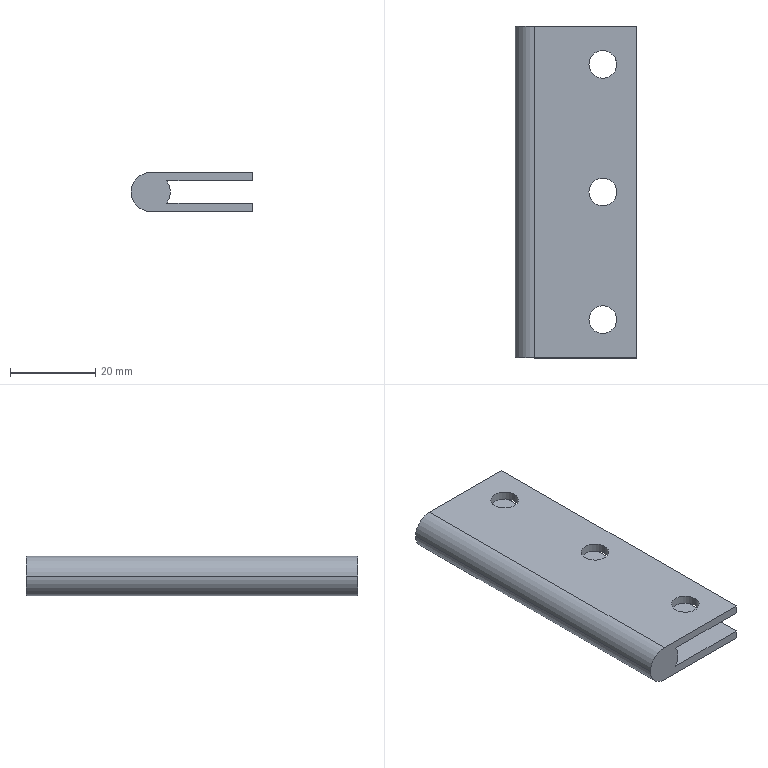Component | SolidWorks | SYM0671-81-200-1_SYMA1-51a_mis_shhpsk6-3-1 | 1 solid | 23 faces | box 28.6 x 78 x 9.2 mm | volume 11443 mm3 | cylinder 15 | plane 8 | commonest cylinder face diameters 6.5 x12 9.2 x3
build123d program:
from build123d import *

# Parameters (mm, degrees)
EXTRUDE1_DEPTH     = 39
SKETCH2_R          = 3.25
CUT_EXTRUDE1_DEPTH = 47.023
LPATTERN1_COUNT    = 3
LPATTERN1_PITCH    = 30


with BuildPart() as part:
    # Sketch1 → Extrude1 (new, symmetric)
    with BuildSketch(Plane(origin=(0, 0, 0), x_dir=(1, 0, 0), z_dir=(0, 1, 0))):
        with BuildLine():
            Line((-4.6, 0), (-4.6, -24))
            Line((-4.6, -24), (-2.6, -24))
            Line((-2.6, -24), (-2.6, -3.795))
            ThreePointArc((-2.6, -3.795), (0, -4.6), (2.6, -3.795))
            Line((2.6, -3.795), (2.6, -24))
            Line((2.6, -24), (4.6, -24))
            Line((4.6, -24), (4.6, 0))
            ThreePointArc((4.6, 0), (0, 4.6), (-4.6, 0))
        make_face()
    extrude(amount=EXTRUDE1_DEPTH, both=True)

    # Sketch2 → Cut-Extrude1 (cut, symmetric)
    with BuildSketch(Plane(origin=(0, 0, 0), x_dir=(0, 0, -1), z_dir=(1, 0, 0))):
        with Locations((-16, 30)):
            Circle(SKETCH2_R)
    cut_extrude1 = extrude(amount=CUT_EXTRUDE1_DEPTH, both=True, mode=Mode.SUBTRACT)

    # LPattern1: Cut-Extrude1 ×3
    with Locations(*[(0, -i * LPATTERN1_PITCH, 0) for i in range(1, LPATTERN1_COUNT)]):
        add(cut_extrude1, mode=Mode.SUBTRACT)


solid = part.part

# Placed as in the assembly
solid = solid.moved(Location((-402.749, 333.143, 1035.118), (0, 90, 0)))
STEP:
#1=COLOUR_RGB('',0.7922,0.8196,0.9333);
#2=FILL_AREA_STYLE_COLOUR('',#1);
#3=FILL_AREA_STYLE('',(#2));
#4=SURFACE_STYLE_FILL_AREA(#3);
#5=SURFACE_SIDE_STYLE('',(#4));
#6=SURFACE_STYLE_USAGE(.BOTH.,#5);
#7=PRESENTATION_STYLE_ASSIGNMENT((#6));
#8=CARTESIAN_POINT('',(-15.098,11.935,40.934));
#9=VERTEX_POINT('',#8);
#10=CARTESIAN_POINT('',(-15.354,11.935,40.934));
#11=VERTEX_POINT('',#10);
#12=CARTESIAN_POINT('',(-15.226,11.935,40.934));
#13=DIRECTION('',(0.,0.,-1.));
#14=DIRECTION('',(-1.,0.,0.));
#15=AXIS2_PLACEMENT_3D('',#12,#13,#14);
#16=CIRCLE('',#15,0.128);
#17=EDGE_CURVE('',#9,#11,#16,.T.);
#18=ORIENTED_EDGE('',*,*,#17,.F.);
#19=CARTESIAN_POINT('',(-15.098,11.935,40.855));
#20=VERTEX_POINT('',#19);
#21=CARTESIAN_POINT('',(-15.098,11.935,40.934));
#22=DIRECTION('',(0.,0.,-1.));
#23=VECTOR('',#22,39.37);
#24=LINE('',#21,#23);
#25=EDGE_CURVE('',#9,#20,#24,.T.);
#26=ORIENTED_EDGE('',*,*,#25,.T.);
#27=CARTESIAN_POINT('',(-15.354,11.935,40.855));
#28=VERTEX_POINT('',#27);
#29=CARTESIAN_POINT('',(-15.226,11.935,40.855));
#30=DIRECTION('',(0.,0.,1.));
#31=DIRECTION('',(1.,0.,0.));
#32=AXIS2_PLACEMENT_3D('',#29,#30,#31);
#33=CIRCLE('',#32,0.128);
#34=EDGE_CURVE('',#28,#20,#33,.T.);
#35=ORIENTED_EDGE('',*,*,#34,.F.);
#36=CARTESIAN_POINT('',(-15.354,11.935,40.934));
#37=DIRECTION('',(0.,0.,-1.));
#38=VECTOR('',#37,39.37);
#39=LINE('',#36,#38);
#40=EDGE_CURVE('',#11,#28,#39,.T.);
#41=ORIENTED_EDGE('',*,*,#40,.F.);
#42=EDGE_LOOP('',(#18,#26,#35,#41));
#43=FACE_OUTER_BOUND('',#42,.T.);
#44=CARTESIAN_POINT('',(-15.226,11.935,40.934));
#45=DIRECTION('',(0.,0.,-1.));
#46=DIRECTION('',(-1.,0.,0.));
#47=AXIS2_PLACEMENT_3D('',#44,#45,#46);
#48=CYLINDRICAL_SURFACE('',#47,0.128);
#49=ADVANCED_FACE('',(#43),#48,.F.);
#50=CARTESIAN_POINT('',(-15.098,11.935,40.65));
#51=VERTEX_POINT('',#50);
#52=CARTESIAN_POINT('',(-15.354,11.935,40.65));
#53=VERTEX_POINT('',#52);
#54=CARTESIAN_POINT('',(-15.226,11.935,40.65));
#55=DIRECTION('',(0.,0.,-1.));
#56=DIRECTION('',(-1.,0.,0.));
#57=AXIS2_PLACEMENT_3D('',#54,#55,#56);
#58=CIRCLE('',#57,0.128);
#59=EDGE_CURVE('',#51,#53,#58,.T.);
#60=ORIENTED_EDGE('',*,*,#59,.F.);
#61=CARTESIAN_POINT('',(-15.098,11.935,40.572));
#62=VERTEX_POINT('',#61);
#63=CARTESIAN_POINT('',(-15.098,11.935,40.934));
#64=DIRECTION('',(0.,0.,-1.));
#65=VECTOR('',#64,39.37);
#66=LINE('',#63,#65);
#67=EDGE_CURVE('',#51,#62,#66,.T.);
#68=ORIENTED_EDGE('',*,*,#67,.T.);
#69=CARTESIAN_POINT('',(-15.354,11.935,40.572));
#70=VERTEX_POINT('',#69);
#71=CARTESIAN_POINT('',(-15.226,11.935,40.572));
#72=DIRECTION('',(0.,0.,-1.));
#73=DIRECTION('',(-1.,0.,0.));
#74=AXIS2_PLACEMENT_3D('',#71,#72,#73);
#75=CIRCLE('',#74,0.128);
#76=EDGE_CURVE('',#62,#70,#75,.T.);
#77=ORIENTED_EDGE('',*,*,#76,.T.);
#78=CARTESIAN_POINT('',(-15.354,11.935,40.934));
#79=DIRECTION('',(0.,0.,-1.));
#80=VECTOR('',#79,39.37);
#81=LINE('',#78,#80);
#82=EDGE_CURVE('',#53,#70,#81,.T.);
#83=ORIENTED_EDGE('',*,*,#82,.F.);
#84=EDGE_LOOP('',(#60,#68,#77,#83));
#85=FACE_OUTER_BOUND('',#84,.T.);
#86=CARTESIAN_POINT('',(-15.226,11.935,40.934));
#87=DIRECTION('',(0.,0.,-1.));
#88=DIRECTION('',(-1.,0.,0.));
#89=AXIS2_PLACEMENT_3D('',#86,#87,#88);
#90=CYLINDRICAL_SURFACE('',#89,0.128);
#91=ADVANCED_FACE('',(#85),#90,.F.);
#92=CARTESIAN_POINT('',(-15.098,13.116,40.934));
#93=VERTEX_POINT('',#92);
#94=CARTESIAN_POINT('',(-15.354,13.116,40.934));
#95=VERTEX_POINT('',#94);
#96=CARTESIAN_POINT('',(-15.226,13.116,40.934));
#97=DIRECTION('',(0.,0.,-1.));
#98=DIRECTION('',(-1.,0.,0.));
#99=AXIS2_PLACEMENT_3D('',#96,#97,#98);
#100=CIRCLE('',#99,0.128);
#101=EDGE_CURVE('',#93,#95,#100,.T.);
#102=ORIENTED_EDGE('',*,*,#101,.F.);
#103=CARTESIAN_POINT('',(-15.098,13.116,40.855));
#104=VERTEX_POINT('',#103);
#105=CARTESIAN_POINT('',(-15.098,13.116,40.934));
#106=DIRECTION('',(0.,0.,-1.));
#107=VECTOR('',#106,39.37);
#108=LINE('',#105,#107);
#109=EDGE_CURVE('',#93,#104,#108,.T.);
#110=ORIENTED_EDGE('',*,*,#109,.T.);
#111=CARTESIAN_POINT('',(-15.354,13.116,40.855));
#112=VERTEX_POINT('',#111);
#113=CARTESIAN_POINT('',(-15.226,13.116,40.855));
#114=DIRECTION('',(0.,0.,1.));
#115=DIRECTION('',(1.,0.,0.));
#116=AXIS2_PLACEMENT_3D('',#113,#114,#115);
#117=CIRCLE('',#116,0.128);
#118=EDGE_CURVE('',#112,#104,#117,.T.);
#119=ORIENTED_EDGE('',*,*,#118,.F.);
#120=CARTESIAN_POINT('',(-15.354,13.116,40.934));
#121=DIRECTION('',(0.,0.,-1.));
#122=VECTOR('',#121,39.37);
#123=LINE('',#120,#122);
#124=EDGE_CURVE('',#95,#112,#123,.T.);
#125=ORIENTED_EDGE('',*,*,#124,.F.);
#126=EDGE_LOOP('',(#102,#110,#119,#125));
#127=FACE_OUTER_BOUND('',#126,.T.);
#128=CARTESIAN_POINT('',(-15.226,13.116,40.934));
#129=DIRECTION('',(0.,0.,-1.));
#130=DIRECTION('',(-1.,0.,0.));
#131=AXIS2_PLACEMENT_3D('',#128,#129,#130);
#132=CYLINDRICAL_SURFACE('',#131,0.128);
#133=ADVANCED_FACE('',(#127),#132,.F.);
#134=CARTESIAN_POINT('',(-15.098,13.116,40.65));
#135=VERTEX_POINT('',#134);
#136=CARTESIAN_POINT('',(-15.354,13.116,40.65));
#137=VERTEX_POINT('',#136);
#138=CARTESIAN_POINT('',(-15.226,13.116,40.65));
#139=DIRECTION('',(0.,0.,-1.));
#140=DIRECTION('',(-1.,0.,0.));
#141=AXIS2_PLACEMENT_3D('',#138,#139,#140);
#142=CIRCLE('',#141,0.128);
#143=EDGE_CURVE('',#135,#137,#142,.T.);
#144=ORIENTED_EDGE('',*,*,#143,.F.);
#145=CARTESIAN_POINT('',(-15.098,13.116,40.572));
#146=VERTEX_POINT('',#145);
#147=CARTESIAN_POINT('',(-15.098,13.116,40.934));
#148=DIRECTION('',(0.,0.,-1.));
#149=VECTOR('',#148,39.37);
#150=LINE('',#147,#149);
#151=EDGE_CURVE('',#135,#146,#150,.T.);
#152=ORIENTED_EDGE('',*,*,#151,.T.);
#153=CARTESIAN_POINT('',(-15.354,13.116,40.572));
#154=VERTEX_POINT('',#153);
#155=CARTESIAN_POINT('',(-15.226,13.116,40.572));
#156=DIRECTION('',(0.,0.,-1.));
#157=DIRECTION('',(-1.,0.,0.));
#158=AXIS2_PLACEMENT_3D('',#155,#156,#157);
#159=CIRCLE('',#158,0.128);
#160=EDGE_CURVE('',#146,#154,#159,.T.);
#161=ORIENTED_EDGE('',*,*,#160,.T.);
#162=CARTESIAN_POINT('',(-15.354,13.116,40.934));
#163=DIRECTION('',(0.,0.,-1.));
#164=VECTOR('',#163,39.37);
#165=LINE('',#162,#164);
#166=EDGE_CURVE('',#137,#154,#165,.T.);
#167=ORIENTED_EDGE('',*,*,#166,.F.);
#168=EDGE_LOOP('',(#144,#152,#161,#167));
#169=FACE_OUTER_BOUND('',#168,.T.);
#170=CARTESIAN_POINT('',(-15.226,13.116,40.934));
#171=DIRECTION('',(0.,0.,-1.));
#172=DIRECTION('',(-1.,0.,0.));
#173=AXIS2_PLACEMENT_3D('',#170,#171,#172);
#174=CYLINDRICAL_SURFACE('',#173,0.128);
#175=ADVANCED_FACE('',(#169),#174,.F.);
#176=CARTESIAN_POINT('',(-15.098,14.297,40.934));
#177=VERTEX_POINT('',#176);
#178=CARTESIAN_POINT('',(-15.354,14.297,40.934));
#179=VERTEX_POINT('',#178);
#180=CARTESIAN_POINT('',(-15.226,14.297,40.934));
#181=DIRECTION('',(0.,0.,-1.));
#182=DIRECTION('',(-1.,0.,0.));
#183=AXIS2_PLACEMENT_3D('',#180,#181,#182);
#184=CIRCLE('',#183,0.128);
#185=EDGE_CURVE('',#177,#179,#184,.T.);
#186=ORIENTED_EDGE('',*,*,#185,.F.);
#187=CARTESIAN_POINT('',(-15.098,14.297,40.855));
#188=VERTEX_POINT('',#187);
#189=CARTESIAN_POINT('',(-15.098,14.297,40.934));
#190=DIRECTION('',(0.,0.,-1.));
#191=VECTOR('',#190,39.37);
#192=LINE('',#189,#191);
#193=EDGE_CURVE('',#177,#188,#192,.T.);
#194=ORIENTED_EDGE('',*,*,#193,.T.);
#195=CARTESIAN_POINT('',(-15.354,14.297,40.855));
#196=VERTEX_POINT('',#195);
#197=CARTESIAN_POINT('',(-15.226,14.297,40.855));
#198=DIRECTION('',(0.,0.,1.));
#199=DIRECTION('',(1.,0.,0.));
#200=AXIS2_PLACEMENT_3D('',#197,#198,#199);
#201=CIRCLE('',#200,0.128);
#202=EDGE_CURVE('',#196,#188,#201,.T.);
#203=ORIENTED_EDGE('',*,*,#202,.F.);
#204=CARTESIAN_POINT('',(-15.354,14.297,40.934));
#205=DIRECTION('',(0.,0.,-1.));
#206=VECTOR('',#205,39.37);
#207=LINE('',#204,#206);
#208=EDGE_CURVE('',#179,#196,#207,.T.);
#209=ORIENTED_EDGE('',*,*,#208,.F.);
#210=EDGE_LOOP('',(#186,#194,#203,#209));
#211=FACE_OUTER_BOUND('',#210,.T.);
#212=CARTESIAN_POINT('',(-15.226,14.297,40.934));
#213=DIRECTION('',(0.,0.,-1.));
#214=DIRECTION('',(-1.,0.,0.));
#215=AXIS2_PLACEMENT_3D('',#212,#213,#214);
#216=CYLINDRICAL_SURFACE('',#215,0.128);
#217=ADVANCED_FACE('',(#211),#216,.F.);
#218=CARTESIAN_POINT('',(-15.098,14.297,40.65));
#219=VERTEX_POINT('',#218);
#220=CARTESIAN_POINT('',(-15.354,14.297,40.65));
#221=VERTEX_POINT('',#220);
#222=CARTESIAN_POINT('',(-15.226,14.297,40.65));
#223=DIRECTION('',(0.,0.,-1.));
#224=DIRECTION('',(-1.,0.,0.));
#225=AXIS2_PLACEMENT_3D('',#222,#223,#224);
#226=CIRCLE('',#225,0.128);
#227=EDGE_CURVE('',#219,#221,#226,.T.);
#228=ORIENTED_EDGE('',*,*,#227,.F.);
#229=CARTESIAN_POINT('',(-15.098,14.297,40.572));
#230=VERTEX_POINT('',#229);
#231=CARTESIAN_POINT('',(-15.098,14.297,40.934));
#232=DIRECTION('',(0.,0.,-1.));
#233=VECTOR('',#232,39.37);
#234=LINE('',#231,#233);
#235=EDGE_CURVE('',#219,#230,#234,.T.);
#236=ORIENTED_EDGE('',*,*,#235,.T.);
#237=CARTESIAN_POINT('',(-15.354,14.297,40.572));
#238=VERTEX_POINT('',#237);
#239=CARTESIAN_POINT('',(-15.226,14.297,40.572));
#240=DIRECTION('',(0.,0.,-1.));
#241=DIRECTION('',(-1.,0.,0.));
#242=AXIS2_PLACEMENT_3D('',#239,#240,#241);
#243=CIRCLE('',#242,0.128);
#244=EDGE_CURVE('',#230,#238,#243,.T.);
#245=ORIENTED_EDGE('',*,*,#244,.T.);
#246=CARTESIAN_POINT('',(-15.354,14.297,40.934));
#247=DIRECTION('',(0.,0.,-1.));
#248=VECTOR('',#247,39.37);
#249=LINE('',#246,#248);
#250=EDGE_CURVE('',#221,#238,#249,.T.);
#251=ORIENTED_EDGE('',*,*,#250,.F.);
#252=EDGE_LOOP('',(#228,#236,#245,#251));
#253=FACE_OUTER_BOUND('',#252,.T.);
#254=CARTESIAN_POINT('',(-15.226,14.297,40.934));
#255=DIRECTION('',(0.,0.,-1.));
#256=DIRECTION('',(-1.,0.,0.));
#257=AXIS2_PLACEMENT_3D('',#254,#255,#256);
#258=CYLINDRICAL_SURFACE('',#257,0.128);
#259=ADVANCED_FACE('',(#253),#258,.F.);
#260=CARTESIAN_POINT('',(-16.037,14.651,40.753));
#261=VERTEX_POINT('',#260);
#262=CARTESIAN_POINT('',(-15.856,14.651,40.934));
#263=VERTEX_POINT('',#262);
#264=CARTESIAN_POINT('',(-15.856,14.651,40.753));
#265=DIRECTION('',(0.,1.,0.));
#266=DIRECTION('',(1.,0.,0.));
#267=AXIS2_PLACEMENT_3D('',#264,#265,#266);
#268=CIRCLE('',#267,0.1811);
#269=EDGE_CURVE('',#261,#263,#268,.T.);
#270=ORIENTED_EDGE('',*,*,#269,.F.);
#271=CARTESIAN_POINT('',(-16.037,11.58,40.753));
#272=VERTEX_POINT('',#271);
#273=CARTESIAN_POINT('',(-16.037,14.651,40.753));
#274=DIRECTION('',(0.,-1.,0.));
#275=VECTOR('',#274,39.37);
#276=LINE('',#273,#275);
#277=EDGE_CURVE('',#261,#272,#276,.T.);
#278=ORIENTED_EDGE('',*,*,#277,.T.);
#279=CARTESIAN_POINT('',(-15.856,11.58,40.934));
#280=VERTEX_POINT('',#279);
#281=CARTESIAN_POINT('',(-15.856,11.58,40.753));
#282=DIRECTION('',(0.,1.,0.));
#283=DIRECTION('',(1.,0.,0.));
#284=AXIS2_PLACEMENT_3D('',#281,#282,#283);
#285=CIRCLE('',#284,0.1811);
#286=EDGE_CURVE('',#272,#280,#285,.T.);
#287=ORIENTED_EDGE('',*,*,#286,.T.);
#288=CARTESIAN_POINT('',(-15.856,14.651,40.934));
#289=DIRECTION('',(0.,-1.,0.));
#290=VECTOR('',#289,39.37);
#291=LINE('',#288,#290);
#292=EDGE_CURVE('',#263,#280,#291,.T.);
#293=ORIENTED_EDGE('',*,*,#292,.F.);
#294=EDGE_LOOP('',(#270,#278,#287,#293));
#295=FACE_OUTER_BOUND('',#294,.T.);
#296=CARTESIAN_POINT('',(-15.856,14.651,40.753));
#297=DIRECTION('',(0.,-1.,0.));
#298=DIRECTION('',(-1.,0.,0.));
#299=AXIS2_PLACEMENT_3D('',#296,#297,#298);
#300=CYLINDRICAL_SURFACE('',#299,0.1811);
#301=ADVANCED_FACE('',(#295),#300,.T.);
#302=ORIENTED_EDGE('',*,*,#277,.F.);
#303=CARTESIAN_POINT('',(-15.856,14.651,40.572));
#304=VERTEX_POINT('',#303);
#305=CARTESIAN_POINT('',(-15.856,14.651,40.753));
#306=DIRECTION('',(0.,1.,0.));
#307=DIRECTION('',(1.,0.,0.));
#308=AXIS2_PLACEMENT_3D('',#305,#306,#307);
#309=CIRCLE('',#308,0.1811);
#310=EDGE_CURVE('',#304,#261,#309,.T.);
#311=ORIENTED_EDGE('',*,*,#310,.F.);
#312=CARTESIAN_POINT('',(-15.856,11.58,40.572));
#313=VERTEX_POINT('',#312);
#314=CARTESIAN_POINT('',(-15.856,14.651,40.572));
#315=DIRECTION('',(0.,-1.,0.));
#316=VECTOR('',#315,39.37);
#317=LINE('',#314,#316);
#318=EDGE_CURVE('',#304,#313,#317,.T.);
#319=ORIENTED_EDGE('',*,*,#318,.T.);
#320=CARTESIAN_POINT('',(-15.856,11.58,40.753));
#321=DIRECTION('',(0.,1.,0.));
#322=DIRECTION('',(1.,0.,0.));
#323=AXIS2_PLACEMENT_3D('',#320,#321,#322);
#324=CIRCLE('',#323,0.1811);
#325=EDGE_CURVE('',#313,#272,#324,.T.);
#326=ORIENTED_EDGE('',*,*,#325,.T.);
#327=EDGE_LOOP('',(#302,#311,#319,#326));
#328=FACE_OUTER_BOUND('',#327,.T.);
#329=CARTESIAN_POINT('',(-15.856,14.651,40.753));
#330=DIRECTION('',(0.,-1.,0.));
#331=DIRECTION('',(-1.,0.,0.));
#332=AXIS2_PLACEMENT_3D('',#329,#330,#331);
#333=CYLINDRICAL_SURFACE('',#332,0.1811);
#334=ADVANCED_FACE('',(#328),#333,.T.);
#335=CARTESIAN_POINT('',(-15.226,11.935,40.934));
#336=DIRECTION('',(0.,0.,-1.));
#337=DIRECTION('',(-1.,0.,0.));
#338=AXIS2_PLACEMENT_3D('',#335,#336,#337);
#339=CIRCLE('',#338,0.128);
#340=EDGE_CURVE('',#11,#9,#339,.T.);
#341=ORIENTED_EDGE('',*,*,#340,.T.);
#342=ORIENTED_EDGE('',*,*,#17,.T.);
#343=EDGE_LOOP('',(#341,#342));
#344=FACE_BOUND('',#343,.T.);
#345=CARTESIAN_POINT('',(-15.226,13.116,40.934));
#346=DIRECTION('',(0.,0.,-1.));
#347=DIRECTION('',(-1.,0.,0.));
#348=AXIS2_PLACEMENT_3D('',#345,#346,#347);
#349=CIRCLE('',#348,0.128);
#350=EDGE_CURVE('',#95,#93,#349,.T.);
#351=ORIENTED_EDGE('',*,*,#350,.T.);
#352=ORIENTED_EDGE('',*,*,#101,.T.);
#353=EDGE_LOOP('',(#351,#352));
#354=FACE_BOUND('',#353,.T.);
#355=CARTESIAN_POINT('',(-15.226,14.297,40.934));
#356=DIRECTION('',(0.,0.,-1.));
#357=DIRECTION('',(-1.,0.,0.));
#358=AXIS2_PLACEMENT_3D('',#355,#356,#357);
#359=CIRCLE('',#358,0.128);
#360=EDGE_CURVE('',#179,#177,#359,.T.);
#361=ORIENTED_EDGE('',*,*,#360,.T.);
#362=ORIENTED_EDGE('',*,*,#185,.T.);
#363=EDGE_LOOP('',(#361,#362));
#364=FACE_BOUND('',#363,.T.);
#365=CARTESIAN_POINT('',(-14.911,11.58,40.934));
#366=VERTEX_POINT('',#365);
#367=CARTESIAN_POINT('',(-15.856,11.58,40.934));
#368=DIRECTION('',(1.,0.,0.));
#369=VECTOR('',#368,39.37);
#370=LINE('',#367,#369);
#371=EDGE_CURVE('',#280,#366,#370,.T.);
#372=ORIENTED_EDGE('',*,*,#371,.T.);
#373=CARTESIAN_POINT('',(-14.911,14.651,40.934));
#374=VERTEX_POINT('',#373);
#375=CARTESIAN_POINT('',(-14.911,14.651,40.934));
#376=DIRECTION('',(0.,-1.,0.));
#377=VECTOR('',#376,39.37);
#378=LINE('',#375,#377);
#379=EDGE_CURVE('',#374,#366,#378,.T.);
#380=ORIENTED_EDGE('',*,*,#379,.F.);
#381=CARTESIAN_POINT('',(-15.856,14.651,40.934));
#382=DIRECTION('',(1.,0.,0.));
#383=VECTOR('',#382,39.37);
#384=LINE('',#381,#383);
#385=EDGE_CURVE('',#263,#374,#384,.T.);
#386=ORIENTED_EDGE('',*,*,#385,.F.);
#387=ORIENTED_EDGE('',*,*,#292,.T.);
#388=EDGE_LOOP('',(#372,#380,#386,#387));
#389=FACE_OUTER_BOUND('',#388,.T.);
#390=CARTESIAN_POINT('',(-15.856,14.651,40.934));
#391=DIRECTION('',(0.,0.,-1.));
#392=DIRECTION('',(-1.,0.,-0.));
#393=AXIS2_PLACEMENT_3D('',#390,#391,#392);
#394=PLANE('',#393);
#395=ADVANCED_FACE('',(#344,#354,#364,#389),#394,.F.);
#396=CARTESIAN_POINT('',(-14.911,11.58,40.855));
#397=VERTEX_POINT('',#396);
#398=CARTESIAN_POINT('',(-14.911,11.58,40.934));
#399=DIRECTION('',(0.,0.,-1.));
#400=VECTOR('',#399,39.37);
#401=LINE('',#398,#400);
#402=EDGE_CURVE('',#366,#397,#401,.T.);
#403=ORIENTED_EDGE('',*,*,#402,.T.);
#404=CARTESIAN_POINT('',(-14.911,14.651,40.855));
#405=VERTEX_POINT('',#404);
#406=CARTESIAN_POINT('',(-14.911,14.651,40.855));
#407=DIRECTION('',(0.,-1.,0.));
#408=VECTOR('',#407,39.37);
#409=LINE('',#406,#408);
#410=EDGE_CURVE('',#405,#397,#409,.T.);
#411=ORIENTED_EDGE('',*,*,#410,.F.);
#412=CARTESIAN_POINT('',(-14.911,14.651,40.934));
#413=DIRECTION('',(0.,0.,-1.));
#414=VECTOR('',#413,39.37);
#415=LINE('',#412,#414);
#416=EDGE_CURVE('',#374,#405,#415,.T.);
#417=ORIENTED_EDGE('',*,*,#416,.F.);
#418=ORIENTED_EDGE('',*,*,#379,.T.);
#419=EDGE_LOOP('',(#403,#411,#417,#418));
#420=FACE_OUTER_BOUND('',#419,.T.);
#421=CARTESIAN_POINT('',(-14.911,14.651,40.934));
#422=DIRECTION('',(-1.,0.,0.));
#423=DIRECTION('',(0.,0.,1.));
#424=AXIS2_PLACEMENT_3D('',#421,#422,#423);
#425=PLANE('',#424);
#426=ADVANCED_FACE('',(#420),#425,.F.);
#427=ORIENTED_EDGE('',*,*,#34,.T.);
#428=CARTESIAN_POINT('',(-15.226,11.935,40.855));
#429=DIRECTION('',(0.,0.,1.));
#430=DIRECTION('',(1.,0.,0.));
#431=AXIS2_PLACEMENT_3D('',#428,#429,#430);
#432=CIRCLE('',#431,0.128);
#433=EDGE_CURVE('',#20,#28,#432,.T.);
#434=ORIENTED_EDGE('',*,*,#433,.T.);
#435=EDGE_LOOP('',(#427,#434));
#436=FACE_BOUND('',#435,.T.);
#437=ORIENTED_EDGE('',*,*,#118,.T.);
#438=CARTESIAN_POINT('',(-15.226,13.116,40.855));
#439=DIRECTION('',(0.,0.,1.));
#440=DIRECTION('',(1.,0.,0.));
#441=AXIS2_PLACEMENT_3D('',#438,#439,#440);
#442=CIRCLE('',#441,0.128);
#443=EDGE_CURVE('',#104,#112,#442,.T.);
#444=ORIENTED_EDGE('',*,*,#443,.T.);
#445=EDGE_LOOP('',(#437,#444));
#446=FACE_BOUND('',#445,.T.);
#447=ORIENTED_EDGE('',*,*,#202,.T.);
#448=CARTESIAN_POINT('',(-15.226,14.297,40.855));
#449=DIRECTION('',(0.,0.,1.));
#450=DIRECTION('',(1.,0.,0.));
#451=AXIS2_PLACEMENT_3D('',#448,#449,#450);
#452=CIRCLE('',#451,0.128);
#453=EDGE_CURVE('',#188,#196,#452,.T.);
#454=ORIENTED_EDGE('',*,*,#453,.T.);
#455=EDGE_LOOP('',(#447,#454));
#456=FACE_BOUND('',#455,.T.);
#457=CARTESIAN_POINT('',(-15.707,11.58,40.855));
#458=VERTEX_POINT('',#457);
#459=CARTESIAN_POINT('',(-14.911,11.58,40.855));
#460=DIRECTION('',(-1.,0.,0.));
#461=VECTOR('',#460,39.37);
#462=LINE('',#459,#461);
#463=EDGE_CURVE('',#397,#458,#462,.T.);
#464=ORIENTED_EDGE('',*,*,#463,.T.);
#465=CARTESIAN_POINT('',(-15.707,14.651,40.855));
#466=VERTEX_POINT('',#465);
#467=CARTESIAN_POINT('',(-15.707,14.651,40.855));
#468=DIRECTION('',(0.,-1.,0.));
#469=VECTOR('',#468,39.37);
#470=LINE('',#467,#469);
#471=EDGE_CURVE('',#466,#458,#470,.T.);
#472=ORIENTED_EDGE('',*,*,#471,.F.);
#473=CARTESIAN_POINT('',(-14.911,14.651,40.855));
#474=DIRECTION('',(-1.,0.,0.));
#475=VECTOR('',#474,39.37);
#476=LINE('',#473,#475);
#477=EDGE_CURVE('',#405,#466,#476,.T.);
#478=ORIENTED_EDGE('',*,*,#477,.F.);
#479=ORIENTED_EDGE('',*,*,#410,.T.);
#480=EDGE_LOOP('',(#464,#472,#478,#479));
#481=FACE_OUTER_BOUND('',#480,.T.);
#482=CARTESIAN_POINT('',(-14.911,14.651,40.855));
#483=DIRECTION('',(0.,0.,1.));
#484=DIRECTION('',(1.,0.,-0.));
#485=AXIS2_PLACEMENT_3D('',#482,#483,#484);
#486=PLANE('',#485);
#487=ADVANCED_FACE('',(#436,#446,#456,#481),#486,.F.);
#488=CARTESIAN_POINT('',(-15.707,11.58,40.65));
#489=VERTEX_POINT('',#488);
#490=CARTESIAN_POINT('',(-15.856,11.58,40.753));
#491=DIRECTION('',(0.,1.,0.));
#492=DIRECTION('',(1.,0.,0.));
#493=AXIS2_PLACEMENT_3D('',#490,#491,#492);
#494=CIRCLE('',#493,0.1811);
#495=EDGE_CURVE('',#458,#489,#494,.T.);
#496=ORIENTED_EDGE('',*,*,#495,.T.);
#497=CARTESIAN_POINT('',(-15.707,14.651,40.65));
#498=VERTEX_POINT('',#497);
#499=CARTESIAN_POINT('',(-15.707,14.651,40.65));
#500=DIRECTION('',(0.,-1.,0.));
#501=VECTOR('',#500,39.37);
#502=LINE('',#499,#501);
#503=EDGE_CURVE('',#498,#489,#502,.T.);
#504=ORIENTED_EDGE('',*,*,#503,.F.);
#505=CARTESIAN_POINT('',(-15.856,14.651,40.753));
#506=DIRECTION('',(0.,1.,0.));
#507=DIRECTION('',(1.,0.,0.));
#508=AXIS2_PLACEMENT_3D('',#505,#506,#507);
#509=CIRCLE('',#508,0.1811);
#510=EDGE_CURVE('',#466,#498,#509,.T.);
#511=ORIENTED_EDGE('',*,*,#510,.F.);
#512=ORIENTED_EDGE('',*,*,#471,.T.);
#513=EDGE_LOOP('',(#496,#504,#511,#512));
#514=FACE_OUTER_BOUND('',#513,.T.);
#515=CARTESIAN_POINT('',(-15.856,14.651,40.753));
#516=DIRECTION('',(0.,-1.,0.));
#517=DIRECTION('',(-1.,0.,0.));
#518=AXIS2_PLACEMENT_3D('',#515,#516,#517);
#519=CYLINDRICAL_SURFACE('',#518,0.1811);
#520=ADVANCED_FACE('',(#514),#519,.T.);
#521=CARTESIAN_POINT('',(-15.226,11.935,40.65));
#522=DIRECTION('',(0.,0.,-1.));
#523=DIRECTION('',(-1.,0.,0.));
#524=AXIS2_PLACEMENT_3D('',#521,#522,#523);
#525=CIRCLE('',#524,0.128);
#526=EDGE_CURVE('',#53,#51,#525,.T.);
#527=ORIENTED_EDGE('',*,*,#526,.T.);
#528=ORIENTED_EDGE('',*,*,#59,.T.);
#529=EDGE_LOOP('',(#527,#528));
#530=FACE_BOUND('',#529,.T.);
#531=CARTESIAN_POINT('',(-15.226,13.116,40.65));
#532=DIRECTION('',(0.,0.,-1.));
#533=DIRECTION('',(-1.,0.,0.));
#534=AXIS2_PLACEMENT_3D('',#531,#532,#533);
#535=CIRCLE('',#534,0.128);
#536=EDGE_CURVE('',#137,#135,#535,.T.);
#537=ORIENTED_EDGE('',*,*,#536,.T.);
#538=ORIENTED_EDGE('',*,*,#143,.T.);
#539=EDGE_LOOP('',(#537,#538));
#540=FACE_BOUND('',#539,.T.);
#541=CARTESIAN_POINT('',(-15.226,14.297,40.65));
#542=DIRECTION('',(0.,0.,-1.));
#543=DIRECTION('',(-1.,0.,0.));
#544=AXIS2_PLACEMENT_3D('',#541,#542,#543);
#545=CIRCLE('',#544,0.128);
#546=EDGE_CURVE('',#221,#219,#545,.T.);
#547=ORIENTED_EDGE('',*,*,#546,.T.);
#548=ORIENTED_EDGE('',*,*,#227,.T.);
#549=EDGE_LOOP('',(#547,#548));
#550=FACE_BOUND('',#549,.T.);
#551=CARTESIAN_POINT('',(-14.911,11.58,40.65));
#552=VERTEX_POINT('',#551);
#553=CARTESIAN_POINT('',(-14.911,11.58,40.65));
#554=DIRECTION('',(1.,0.,0.));
#555=VECTOR('',#554,39.37);
#556=LINE('',#553,#555);
#557=EDGE_CURVE('',#489,#552,#556,.T.);
#558=ORIENTED_EDGE('',*,*,#557,.T.);
#559=CARTESIAN_POINT('',(-14.911,14.651,40.65));
#560=VERTEX_POINT('',#559);
#561=CARTESIAN_POINT('',(-14.911,14.651,40.65));
#562=DIRECTION('',(0.,-1.,0.));
#563=VECTOR('',#562,39.37);
#564=LINE('',#561,#563);
#565=EDGE_CURVE('',#560,#552,#564,.T.);
#566=ORIENTED_EDGE('',*,*,#565,.F.);
#567=CARTESIAN_POINT('',(-14.911,14.651,40.65));
#568=DIRECTION('',(1.,0.,0.));
#569=VECTOR('',#568,39.37);
#570=LINE('',#567,#569);
#571=EDGE_CURVE('',#498,#560,#570,.T.);
#572=ORIENTED_EDGE('',*,*,#571,.F.);
#573=ORIENTED_EDGE('',*,*,#503,.T.);
#574=EDGE_LOOP('',(#558,#566,#572,#573));
#575=FACE_OUTER_BOUND('',#574,.T.);
#576=CARTESIAN_POINT('',(-14.911,14.651,40.65));
#577=DIRECTION('',(0.,0.,-1.));
#578=DIRECTION('',(-1.,0.,-0.));
#579=AXIS2_PLACEMENT_3D('',#576,#577,#578);
#580=PLANE('',#579);
#581=ADVANCED_FACE('',(#530,#540,#550,#575),#580,.F.);
#582=CARTESIAN_POINT('',(-14.911,11.58,40.572));
#583=VERTEX_POINT('',#582);
#584=CARTESIAN_POINT('',(-14.911,11.58,40.572));
#585=DIRECTION('',(0.,0.,-1.));
#586=VECTOR('',#585,39.37);
#587=LINE('',#584,#586);
#588=EDGE_CURVE('',#552,#583,#587,.T.);
#589=ORIENTED_EDGE('',*,*,#588,.T.);
#590=CARTESIAN_POINT('',(-14.911,14.651,40.572));
#591=VERTEX_POINT('',#590);
#592=CARTESIAN_POINT('',(-14.911,14.651,40.572));
#593=DIRECTION('',(0.,-1.,0.));
#594=VECTOR('',#593,39.37);
#595=LINE('',#592,#594);
#596=EDGE_CURVE('',#591,#583,#595,.T.);
#597=ORIENTED_EDGE('',*,*,#596,.F.);
#598=CARTESIAN_POINT('',(-14.911,14.651,40.572));
#599=DIRECTION('',(0.,0.,-1.));
#600=VECTOR('',#599,39.37);
#601=LINE('',#598,#600);
#602=EDGE_CURVE('',#560,#591,#601,.T.);
#603=ORIENTED_EDGE('',*,*,#602,.F.);
#604=ORIENTED_EDGE('',*,*,#565,.T.);
#605=EDGE_LOOP('',(#589,#597,#603,#604));
#606=FACE_OUTER_BOUND('',#605,.T.);
#607=CARTESIAN_POINT('',(-14.911,14.651,40.572));
#608=DIRECTION('',(-1.,0.,0.));
#609=DIRECTION('',(0.,0.,1.));
#610=AXIS2_PLACEMENT_3D('',#607,#608,#609);
#611=PLANE('',#610);
#612=ADVANCED_FACE('',(#606),#611,.F.);
#613=CARTESIAN_POINT('',(-15.226,11.935,40.572));
#614=DIRECTION('',(0.,0.,-1.));
#615=DIRECTION('',(-1.,0.,0.));
#616=AXIS2_PLACEMENT_3D('',#613,#614,#615);
#617=CIRCLE('',#616,0.128);
#618=EDGE_CURVE('',#70,#62,#617,.T.);
#619=ORIENTED_EDGE('',*,*,#618,.F.);
#620=ORIENTED_EDGE('',*,*,#76,.F.);
#621=EDGE_LOOP('',(#619,#620));
#622=FACE_BOUND('',#621,.T.);
#623=CARTESIAN_POINT('',(-15.226,13.116,40.572));
#624=DIRECTION('',(0.,0.,-1.));
#625=DIRECTION('',(-1.,0.,0.));
#626=AXIS2_PLACEMENT_3D('',#623,#624,#625);
#627=CIRCLE('',#626,0.128);
#628=EDGE_CURVE('',#154,#146,#627,.T.);
#629=ORIENTED_EDGE('',*,*,#628,.F.);
#630=ORIENTED_EDGE('',*,*,#160,.F.);
#631=EDGE_LOOP('',(#629,#630));
#632=FACE_BOUND('',#631,.T.);
#633=CARTESIAN_POINT('',(-15.226,14.297,40.572));
#634=DIRECTION('',(0.,0.,-1.));
#635=DIRECTION('',(-1.,0.,0.));
#636=AXIS2_PLACEMENT_3D('',#633,#634,#635);
#637=CIRCLE('',#636,0.128);
#638=EDGE_CURVE('',#238,#230,#637,.T.);
#639=ORIENTED_EDGE('',*,*,#638,.F.);
#640=ORIENTED_EDGE('',*,*,#244,.F.);
#641=EDGE_LOOP('',(#639,#640));
#642=FACE_BOUND('',#641,.T.);
#643=CARTESIAN_POINT('',(-15.856,11.58,40.572));
#644=DIRECTION('',(-1.,0.,0.));
#645=VECTOR('',#644,39.37);
#646=LINE('',#643,#645);
#647=EDGE_CURVE('',#583,#313,#646,.T.);
#648=ORIENTED_EDGE('',*,*,#647,.T.);
#649=ORIENTED_EDGE('',*,*,#318,.F.);
#650=CARTESIAN_POINT('',(-15.856,14.651,40.572));
#651=DIRECTION('',(-1.,0.,0.));
#652=VECTOR('',#651,39.37);
#653=LINE('',#650,#652);
#654=EDGE_CURVE('',#591,#304,#653,.T.);
#655=ORIENTED_EDGE('',*,*,#654,.F.);
#656=ORIENTED_EDGE('',*,*,#596,.T.);
#657=EDGE_LOOP('',(#648,#649,#655,#656));
#658=FACE_OUTER_BOUND('',#657,.T.);
#659=CARTESIAN_POINT('',(-15.856,14.651,40.572));
#660=DIRECTION('',(0.,0.,1.));
#661=DIRECTION('',(1.,0.,-0.));
#662=AXIS2_PLACEMENT_3D('',#659,#660,#661);
#663=PLANE('',#662);
#664=ADVANCED_FACE('',(#622,#632,#642,#658),#663,.F.);
#665=ORIENTED_EDGE('',*,*,#310,.T.);
#666=ORIENTED_EDGE('',*,*,#269,.T.);
#667=ORIENTED_EDGE('',*,*,#385,.T.);
#668=ORIENTED_EDGE('',*,*,#416,.T.);
#669=ORIENTED_EDGE('',*,*,#477,.T.);
#670=ORIENTED_EDGE('',*,*,#510,.T.);
#671=ORIENTED_EDGE('',*,*,#571,.T.);
#672=ORIENTED_EDGE('',*,*,#602,.T.);
#673=ORIENTED_EDGE('',*,*,#654,.T.);
#674=EDGE_LOOP('',(#665,#666,#667,#668,#669,#670,#671,#672,#673));
#675=FACE_OUTER_BOUND('',#674,.T.);
#676=CARTESIAN_POINT('',(-15.856,14.651,40.753));
#677=DIRECTION('',(0.,1.,0.));
#678=DIRECTION('',(1.,0.,0.));
#679=AXIS2_PLACEMENT_3D('',#676,#677,#678);
#680=PLANE('',#679);
#681=ADVANCED_FACE('',(#675),#680,.T.);
#682=ORIENTED_EDGE('',*,*,#325,.F.);
#683=ORIENTED_EDGE('',*,*,#647,.F.);
#684=ORIENTED_EDGE('',*,*,#588,.F.);
#685=ORIENTED_EDGE('',*,*,#557,.F.);
#686=ORIENTED_EDGE('',*,*,#495,.F.);
#687=ORIENTED_EDGE('',*,*,#463,.F.);
#688=ORIENTED_EDGE('',*,*,#402,.F.);
#689=ORIENTED_EDGE('',*,*,#371,.F.);
#690=ORIENTED_EDGE('',*,*,#286,.F.);
#691=EDGE_LOOP('',(#682,#683,#684,#685,#686,#687,#688,#689,#690));
#692=FACE_OUTER_BOUND('',#691,.T.);
#693=CARTESIAN_POINT('',(-15.856,11.58,40.753));
#694=DIRECTION('',(0.,1.,0.));
#695=DIRECTION('',(1.,0.,0.));
#696=AXIS2_PLACEMENT_3D('',#693,#694,#695);
#697=PLANE('',#696);
#698=ADVANCED_FACE('',(#692),#697,.F.);
#699=ORIENTED_EDGE('',*,*,#235,.F.);
#700=ORIENTED_EDGE('',*,*,#546,.F.);
#701=ORIENTED_EDGE('',*,*,#250,.T.);
#702=ORIENTED_EDGE('',*,*,#638,.T.);
#703=EDGE_LOOP('',(#699,#700,#701,#702));
#704=FACE_OUTER_BOUND('',#703,.T.);
#705=CARTESIAN_POINT('',(-15.226,14.297,40.934));
#706=DIRECTION('',(0.,0.,-1.));
#707=DIRECTION('',(-1.,0.,0.));
#708=AXIS2_PLACEMENT_3D('',#705,#706,#707);
#709=CYLINDRICAL_SURFACE('',#708,0.128);
#710=ADVANCED_FACE('',(#704),#709,.F.);
#711=ORIENTED_EDGE('',*,*,#193,.F.);
#712=ORIENTED_EDGE('',*,*,#360,.F.);
#713=ORIENTED_EDGE('',*,*,#208,.T.);
#714=ORIENTED_EDGE('',*,*,#453,.F.);
#715=EDGE_LOOP('',(#711,#712,#713,#714));
#716=FACE_OUTER_BOUND('',#715,.T.);
#717=CARTESIAN_POINT('',(-15.226,14.297,40.934));
#718=DIRECTION('',(0.,0.,-1.));
#719=DIRECTION('',(-1.,0.,0.));
#720=AXIS2_PLACEMENT_3D('',#717,#718,#719);
#721=CYLINDRICAL_SURFACE('',#720,0.128);
#722=ADVANCED_FACE('',(#716),#721,.F.);
#723=ORIENTED_EDGE('',*,*,#151,.F.);
#724=ORIENTED_EDGE('',*,*,#536,.F.);
#725=ORIENTED_EDGE('',*,*,#166,.T.);
#726=ORIENTED_EDGE('',*,*,#628,.T.);
#727=EDGE_LOOP('',(#723,#724,#725,#726));
#728=FACE_OUTER_BOUND('',#727,.T.);
#729=CARTESIAN_POINT('',(-15.226,13.116,40.934));
#730=DIRECTION('',(0.,0.,-1.));
#731=DIRECTION('',(-1.,0.,0.));
#732=AXIS2_PLACEMENT_3D('',#729,#730,#731);
#733=CYLINDRICAL_SURFACE('',#732,0.128);
#734=ADVANCED_FACE('',(#728),#733,.F.);
#735=ORIENTED_EDGE('',*,*,#109,.F.);
#736=ORIENTED_EDGE('',*,*,#350,.F.);
#737=ORIENTED_EDGE('',*,*,#124,.T.);
#738=ORIENTED_EDGE('',*,*,#443,.F.);
#739=EDGE_LOOP('',(#735,#736,#737,#738));
#740=FACE_OUTER_BOUND('',#739,.T.);
#741=CARTESIAN_POINT('',(-15.226,13.116,40.934));
#742=DIRECTION('',(0.,0.,-1.));
#743=DIRECTION('',(-1.,0.,0.));
#744=AXIS2_PLACEMENT_3D('',#741,#742,#743);
#745=CYLINDRICAL_SURFACE('',#744,0.128);
#746=ADVANCED_FACE('',(#740),#745,.F.);
#747=ORIENTED_EDGE('',*,*,#67,.F.);
#748=ORIENTED_EDGE('',*,*,#526,.F.);
#749=ORIENTED_EDGE('',*,*,#82,.T.);
#750=ORIENTED_EDGE('',*,*,#618,.T.);
#751=EDGE_LOOP('',(#747,#748,#749,#750));
#752=FACE_OUTER_BOUND('',#751,.T.);
#753=CARTESIAN_POINT('',(-15.226,11.935,40.934));
#754=DIRECTION('',(0.,0.,-1.));
#755=DIRECTION('',(-1.,0.,0.));
#756=AXIS2_PLACEMENT_3D('',#753,#754,#755);
#757=CYLINDRICAL_SURFACE('',#756,0.128);
#758=ADVANCED_FACE('',(#752),#757,.F.);
#759=ORIENTED_EDGE('',*,*,#25,.F.);
#760=ORIENTED_EDGE('',*,*,#340,.F.);
#761=ORIENTED_EDGE('',*,*,#40,.T.);
#762=ORIENTED_EDGE('',*,*,#433,.F.);
#763=EDGE_LOOP('',(#759,#760,#761,#762));
#764=FACE_OUTER_BOUND('',#763,.T.);
#765=CARTESIAN_POINT('',(-15.226,11.935,40.934));
#766=DIRECTION('',(0.,0.,-1.));
#767=DIRECTION('',(-1.,0.,0.));
#768=AXIS2_PLACEMENT_3D('',#765,#766,#767);
#769=CYLINDRICAL_SURFACE('',#768,0.128);
#770=ADVANCED_FACE('',(#764),#769,.F.);
#771=CLOSED_SHELL('',(#49,#91,#133,#175,#217,#259,#301,#334,#395,#426,#487,#520,#581,#612,#664,#681,#698,#710,#722,#734,#746,#758,#770));
#772=MANIFOLD_SOLID_BREP('',#771);
#773=STYLED_ITEM('',(#7),#772);
#774=(LENGTH_UNIT()NAMED_UNIT(*)SI_UNIT($,.METRE.));
#775=LENGTH_MEASURE_WITH_UNIT(LENGTH_MEASURE(0.0254),#774);
#776=DIMENSIONAL_EXPONENTS(1.,0.,0.,0.,0.,0.,0.);
#777=(CONVERSION_BASED_UNIT('',#775)LENGTH_UNIT()NAMED_UNIT(#776));
#778=UNCERTAINTY_MEASURE_WITH_UNIT(LENGTH_MEASURE(0.00001),#777,'','');
#779=(NAMED_UNIT(*)PLANE_ANGLE_UNIT()SI_UNIT($,.RADIAN.));
#780=(NAMED_UNIT(*)SI_UNIT($,.STERADIAN.)SOLID_ANGLE_UNIT());
#781=(GEOMETRIC_REPRESENTATION_CONTEXT(3)GLOBAL_UNCERTAINTY_ASSIGNED_CONTEXT((#778))GLOBAL_UNIT_ASSIGNED_CONTEXT((#777,#779,#780))REPRESENTATION_CONTEXT('',''));
#782=MECHANICAL_DESIGN_GEOMETRIC_PRESENTATION_REPRESENTATION('',(#773),#781);
#783=CARTESIAN_POINT('',(0.,0.,0.));
#784=DIRECTION('',(0.,0.,1.));
#785=DIRECTION('',(1.,0.,0.));
#786=AXIS2_PLACEMENT_3D('',#783,#784,#785);
#787=(LENGTH_UNIT()NAMED_UNIT(*)SI_UNIT($,.METRE.));
#788=LENGTH_MEASURE_WITH_UNIT(LENGTH_MEASURE(0.0254),#787);
#789=DIMENSIONAL_EXPONENTS(1.,0.,0.,0.,0.,0.,0.);
#790=(CONVERSION_BASED_UNIT('',#788)LENGTH_UNIT()NAMED_UNIT(#789));
#791=UNCERTAINTY_MEASURE_WITH_UNIT(LENGTH_MEASURE(0.00001),#790,'','');
#792=(NAMED_UNIT(*)PLANE_ANGLE_UNIT()SI_UNIT($,.RADIAN.));
#793=(NAMED_UNIT(*)SI_UNIT($,.STERADIAN.)SOLID_ANGLE_UNIT());
#794=(GEOMETRIC_REPRESENTATION_CONTEXT(3)GLOBAL_UNCERTAINTY_ASSIGNED_CONTEXT((#791))GLOBAL_UNIT_ASSIGNED_CONTEXT((#790,#792,#793))REPRESENTATION_CONTEXT('',''));
#795=ADVANCED_BREP_SHAPE_REPRESENTATION('',(#772,#786),#794);
#796=PRESENTATION_LAYER_ASSIGNMENT('','',(#773));